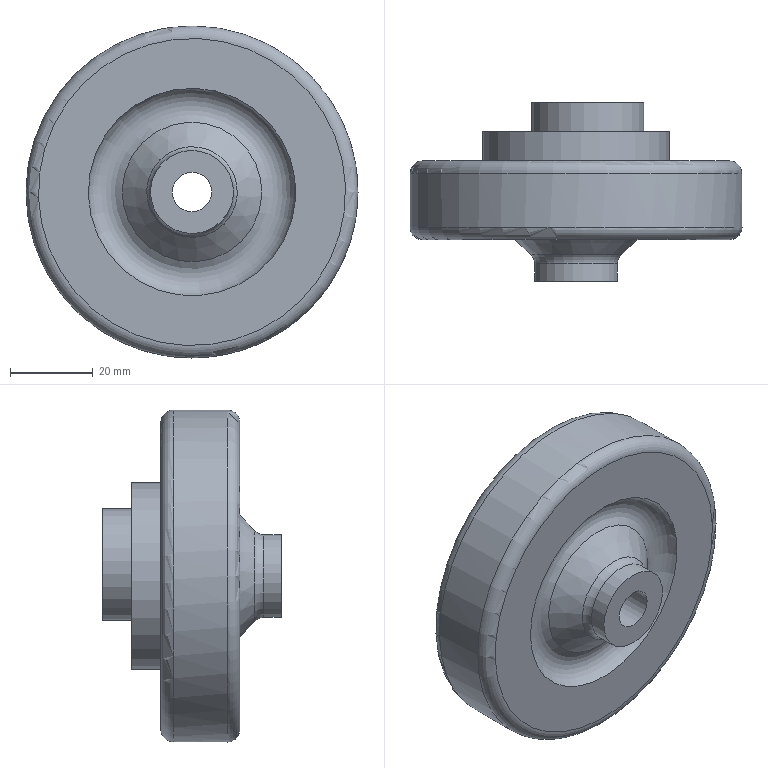Component | NX | FLYWHEEL | 1 solid | 17 faces | volume 104281 mm3 | plane 6 | cylinder 6 | torus 4 | cone 1 | commonest cylinder face diameters 80 x1 45 x1 27 x1 20 x1 9.5 x1 17 x1